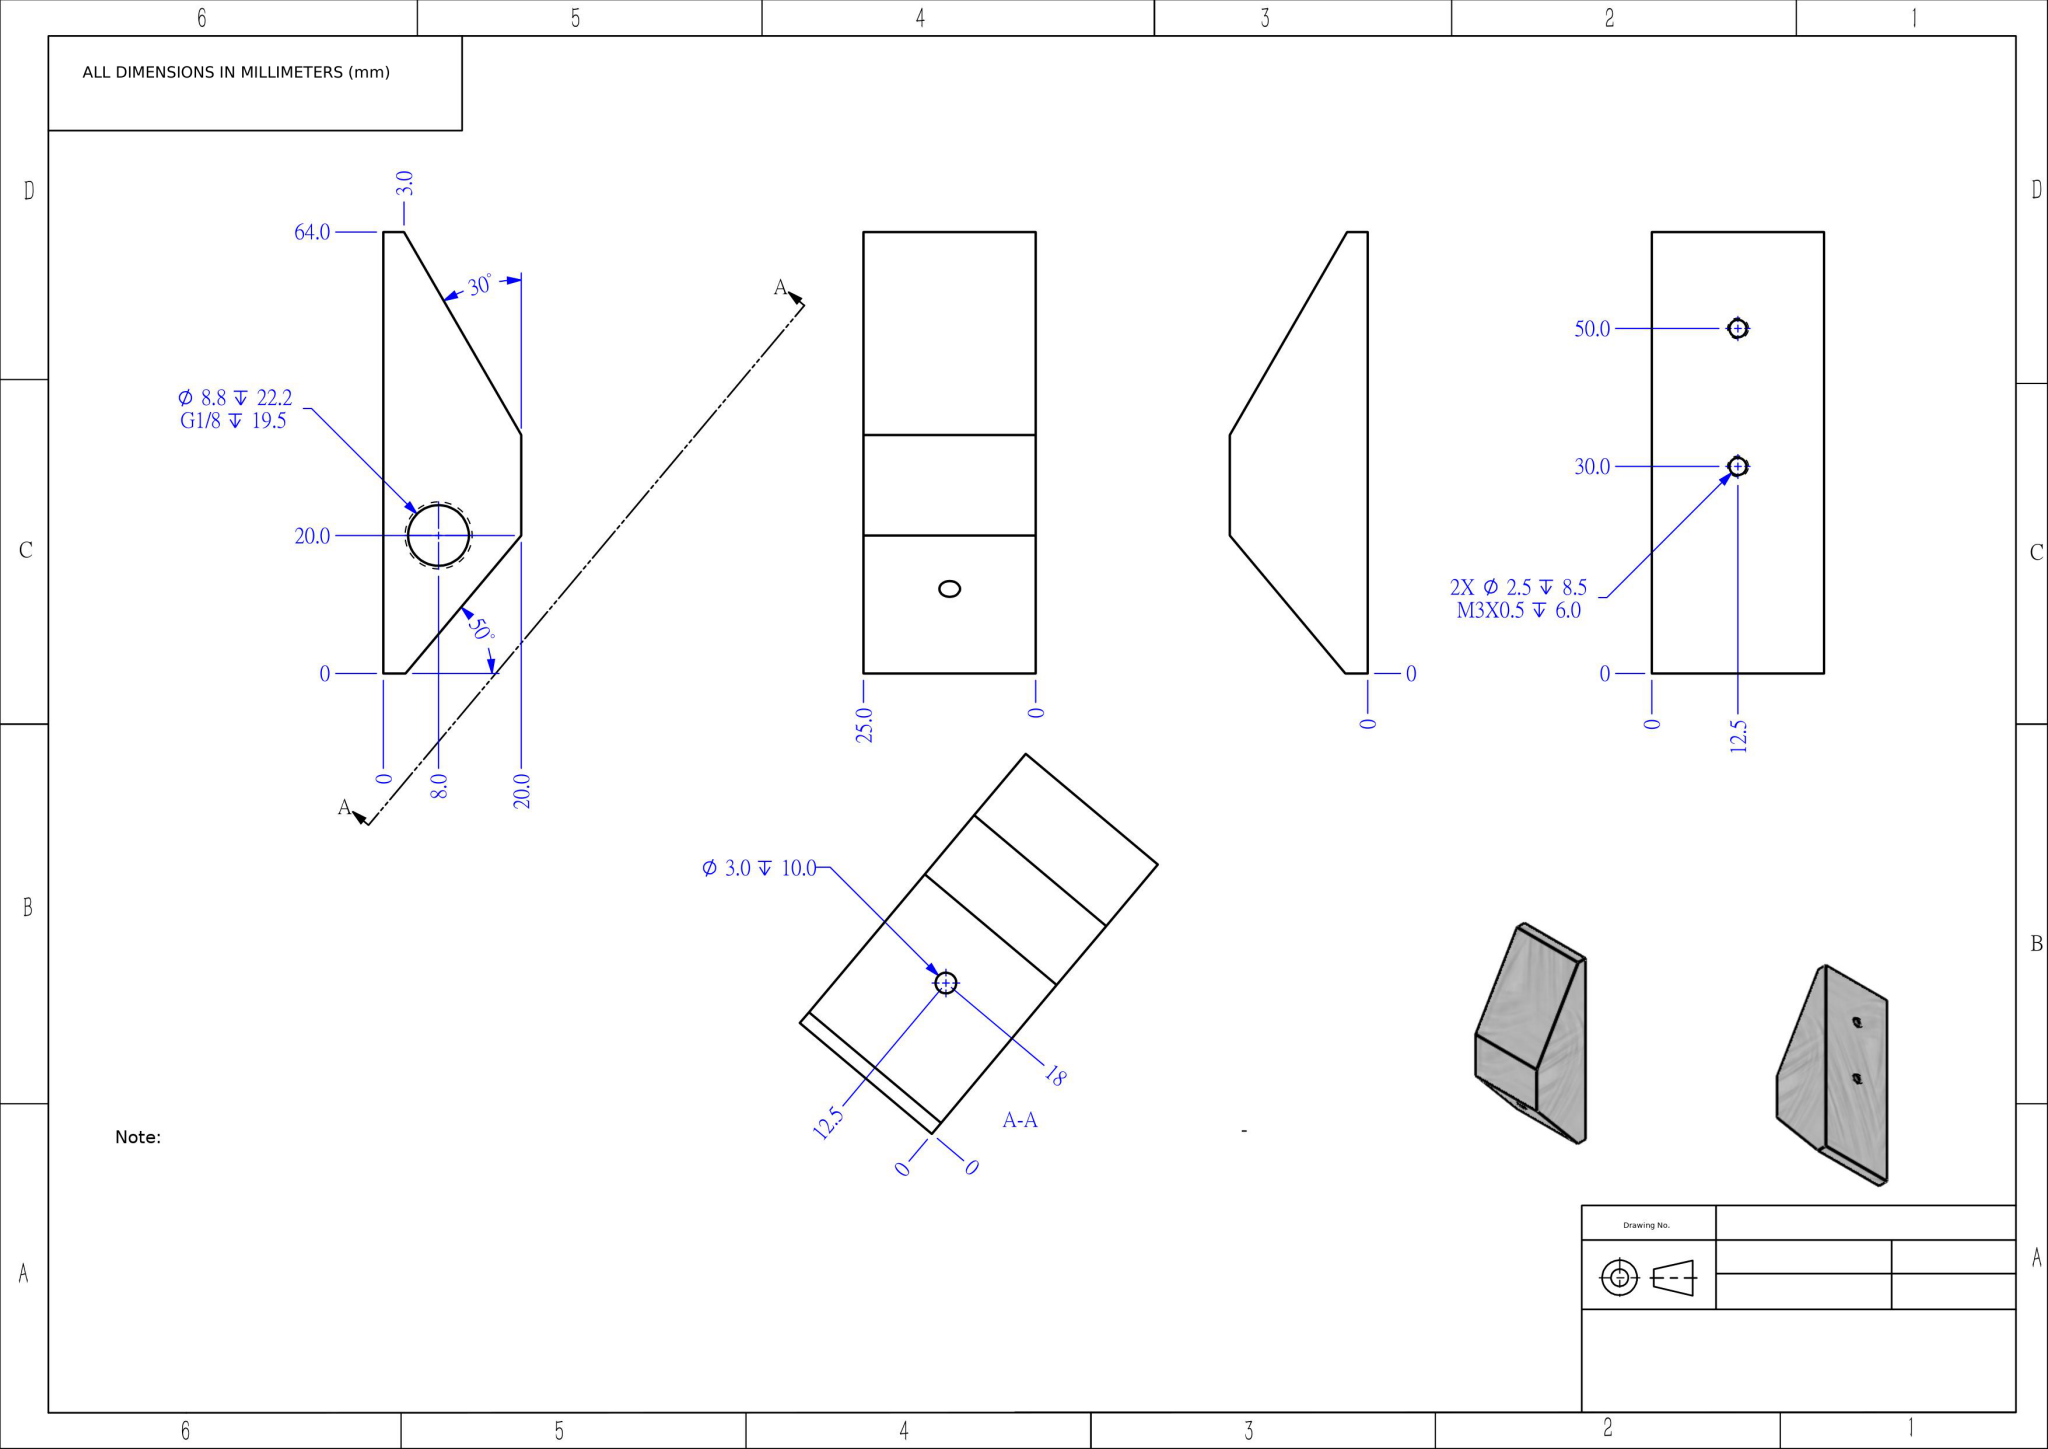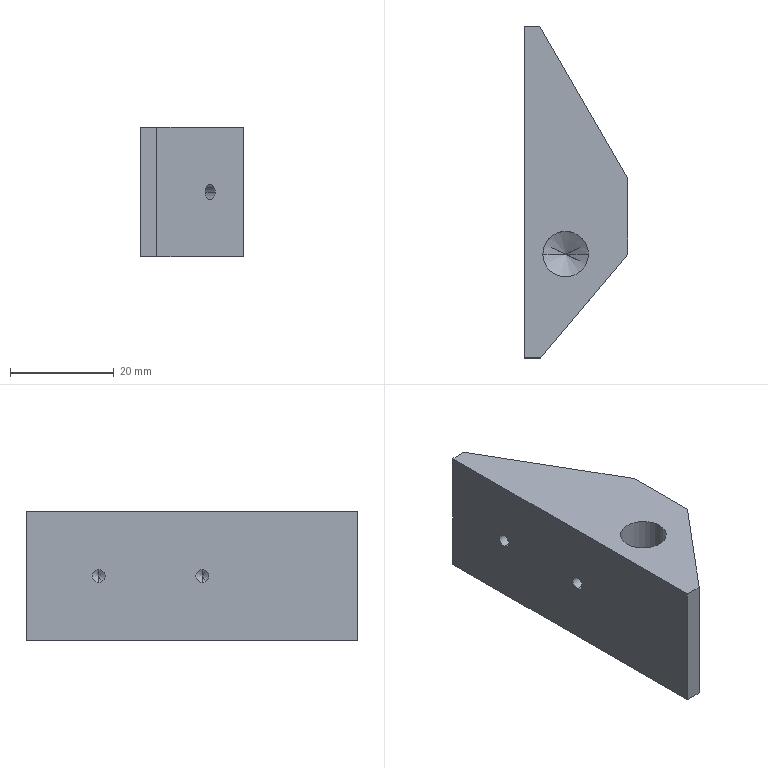Part | NX | mm | 1 solid | 22 faces | box 20 x 64 x 25 mm | volume 20019 mm3 | cylinder 8 | plane 8 | cone 6 | commonest cylinder face diameters 2.5 x4 8.8 x2 3 x2
STEP:
#1=COLOUR_RGB('',1.,1.,1.);
#2=FILL_AREA_STYLE_COLOUR('',#1);
#3=FILL_AREA_STYLE('',(#2));
#4=SURFACE_STYLE_FILL_AREA(#3);
#5=SURFACE_SIDE_STYLE('',(#4));
#6=SURFACE_STYLE_USAGE(.BOTH.,#5);
#7=PRESENTATION_STYLE_ASSIGNMENT((#6));
#8=CARTESIAN_POINT('',(-1.5,18.,11.25));
#9=VERTEX_POINT('',#8);
#10=CARTESIAN_POINT('',(-1.5,18.,13.75));
#11=VERTEX_POINT('',#10);
#12=CARTESIAN_POINT('',(-1.5,18.,12.5));
#13=DIRECTION('',(-1.,0.,0.));
#14=DIRECTION('',(0.,0.,1.));
#15=AXIS2_PLACEMENT_3D('',#12,#13,#14);
#16=CIRCLE('',#15,1.25);
#17=EDGE_CURVE('',#9,#11,#16,.T.);
#18=ORIENTED_EDGE('',*,*,#17,.F.);
#19=CARTESIAN_POINT('',(-10.,18.,11.25));
#20=VERTEX_POINT('',#19);
#21=CARTESIAN_POINT('',(-10.,18.,11.25));
#22=DIRECTION('',(-1.,0.,0.));
#23=VECTOR('',#22,1000.);
#24=LINE('',#21,#23);
#25=EDGE_CURVE('',#9,#20,#24,.T.);
#26=ORIENTED_EDGE('',*,*,#25,.T.);
#27=CARTESIAN_POINT('',(-10.,18.,13.75));
#28=VERTEX_POINT('',#27);
#29=CARTESIAN_POINT('',(-10.,18.,12.5));
#30=DIRECTION('',(-1.,0.,0.));
#31=DIRECTION('',(0.,0.,1.));
#32=AXIS2_PLACEMENT_3D('',#29,#30,#31);
#33=CIRCLE('',#32,1.25);
#34=EDGE_CURVE('',#20,#28,#33,.T.);
#35=ORIENTED_EDGE('',*,*,#34,.T.);
#36=CARTESIAN_POINT('',(-10.,18.,13.75));
#37=DIRECTION('',(-1.,0.,0.));
#38=VECTOR('',#37,1000.);
#39=LINE('',#36,#38);
#40=EDGE_CURVE('',#11,#28,#39,.T.);
#41=ORIENTED_EDGE('',*,*,#40,.F.);
#42=EDGE_LOOP('',(#18,#26,#35,#41));
#43=FACE_OUTER_BOUND('',#42,.T.);
#44=CARTESIAN_POINT('',(-10.,18.,12.5));
#45=DIRECTION('',(-1.,0.,0.));
#46=DIRECTION('',(0.,0.,1.));
#47=AXIS2_PLACEMENT_3D('',#44,#45,#46);
#48=CYLINDRICAL_SURFACE('',#47,1.25);
#49=ADVANCED_FACE('',(#43),#48,.F.);
#50=CARTESIAN_POINT('',(-0.7489,18.,12.5));
#51=VERTEX_POINT('',#50);
#52=CARTESIAN_POINT('',(-1.5,18.,13.75));
#53=DIRECTION('',(-0.515,0.,0.8572));
#54=VECTOR('',#53,1000.);
#55=LINE('',#52,#54);
#56=EDGE_CURVE('',#51,#11,#55,.T.);
#57=ORIENTED_EDGE('',*,*,#56,.F.);
#58=CARTESIAN_POINT('',(-1.5,18.,11.25));
#59=DIRECTION('',(-0.515,0.,-0.8572));
#60=VECTOR('',#59,1000.);
#61=LINE('',#58,#60);
#62=EDGE_CURVE('',#51,#9,#61,.T.);
#63=ORIENTED_EDGE('',*,*,#62,.T.);
#64=ORIENTED_EDGE('',*,*,#17,.T.);
#65=EDGE_LOOP('',(#57,#63,#64));
#66=FACE_OUTER_BOUND('',#65,.T.);
#67=CARTESIAN_POINT('',(-1.5,18.,12.5));
#68=DIRECTION('',(-1.,0.,0.));
#69=DIRECTION('',(0.,0.,1.));
#70=AXIS2_PLACEMENT_3D('',#67,#68,#69);
#71=CONICAL_SURFACE('',#70,1.25,1.03);
#72=ADVANCED_FACE('',(#66),#71,.F.);
#73=CARTESIAN_POINT('',(-1.5,-2.,11.25));
#74=VERTEX_POINT('',#73);
#75=CARTESIAN_POINT('',(-1.5,-2.,13.75));
#76=VERTEX_POINT('',#75);
#77=CARTESIAN_POINT('',(-1.5,-2.,12.5));
#78=DIRECTION('',(-1.,0.,0.));
#79=DIRECTION('',(0.,0.,1.));
#80=AXIS2_PLACEMENT_3D('',#77,#78,#79);
#81=CIRCLE('',#80,1.25);
#82=EDGE_CURVE('',#74,#76,#81,.T.);
#83=ORIENTED_EDGE('',*,*,#82,.F.);
#84=CARTESIAN_POINT('',(-10.,-2.,11.25));
#85=VERTEX_POINT('',#84);
#86=CARTESIAN_POINT('',(-10.,-2.,11.25));
#87=DIRECTION('',(-1.,0.,0.));
#88=VECTOR('',#87,1000.);
#89=LINE('',#86,#88);
#90=EDGE_CURVE('',#74,#85,#89,.T.);
#91=ORIENTED_EDGE('',*,*,#90,.T.);
#92=CARTESIAN_POINT('',(-10.,-2.,13.75));
#93=VERTEX_POINT('',#92);
#94=CARTESIAN_POINT('',(-10.,-2.,12.5));
#95=DIRECTION('',(-1.,0.,0.));
#96=DIRECTION('',(0.,0.,1.));
#97=AXIS2_PLACEMENT_3D('',#94,#95,#96);
#98=CIRCLE('',#97,1.25);
#99=EDGE_CURVE('',#85,#93,#98,.T.);
#100=ORIENTED_EDGE('',*,*,#99,.T.);
#101=CARTESIAN_POINT('',(-10.,-2.,13.75));
#102=DIRECTION('',(-1.,0.,0.));
#103=VECTOR('',#102,1000.);
#104=LINE('',#101,#103);
#105=EDGE_CURVE('',#76,#93,#104,.T.);
#106=ORIENTED_EDGE('',*,*,#105,.F.);
#107=EDGE_LOOP('',(#83,#91,#100,#106));
#108=FACE_OUTER_BOUND('',#107,.T.);
#109=CARTESIAN_POINT('',(-10.,-2.,12.5));
#110=DIRECTION('',(-1.,0.,0.));
#111=DIRECTION('',(0.,0.,1.));
#112=AXIS2_PLACEMENT_3D('',#109,#110,#111);
#113=CYLINDRICAL_SURFACE('',#112,1.25);
#114=ADVANCED_FACE('',(#108),#113,.F.);
#115=CARTESIAN_POINT('',(-0.7489,-2.,12.5));
#116=VERTEX_POINT('',#115);
#117=CARTESIAN_POINT('',(-1.5,-2.,13.75));
#118=DIRECTION('',(-0.515,0.,0.8572));
#119=VECTOR('',#118,1000.);
#120=LINE('',#117,#119);
#121=EDGE_CURVE('',#116,#76,#120,.T.);
#122=ORIENTED_EDGE('',*,*,#121,.F.);
#123=CARTESIAN_POINT('',(-1.5,-2.,11.25));
#124=DIRECTION('',(-0.515,0.,-0.8572));
#125=VECTOR('',#124,1000.);
#126=LINE('',#123,#125);
#127=EDGE_CURVE('',#116,#74,#126,.T.);
#128=ORIENTED_EDGE('',*,*,#127,.T.);
#129=ORIENTED_EDGE('',*,*,#82,.T.);
#130=EDGE_LOOP('',(#122,#128,#129));
#131=FACE_OUTER_BOUND('',#130,.T.);
#132=CARTESIAN_POINT('',(-1.5,-2.,12.5));
#133=DIRECTION('',(-1.,0.,0.));
#134=DIRECTION('',(0.,0.,1.));
#135=AXIS2_PLACEMENT_3D('',#132,#133,#134);
#136=CONICAL_SURFACE('',#135,1.25,1.03);
#137=ADVANCED_FACE('',(#131),#136,.F.);
#138=CARTESIAN_POINT('',(-2.,-12.,0.1792));
#139=VERTEX_POINT('',#138);
#140=CARTESIAN_POINT('',(2.4,-12.,2.823));
#141=VERTEX_POINT('',#140);
#142=CARTESIAN_POINT('',(2.4,-12.,2.823));
#143=DIRECTION('',(0.8572,0.,0.515));
#144=VECTOR('',#143,1000.);
#145=LINE('',#142,#144);
#146=EDGE_CURVE('',#139,#141,#145,.T.);
#147=ORIENTED_EDGE('',*,*,#146,.F.);
#148=CARTESIAN_POINT('',(-6.4,-12.,2.823));
#149=VERTEX_POINT('',#148);
#150=CARTESIAN_POINT('',(-6.4,-12.,2.823));
#151=DIRECTION('',(-0.8572,0.,0.515));
#152=VECTOR('',#151,1000.);
#153=LINE('',#150,#152);
#154=EDGE_CURVE('',#139,#149,#153,.T.);
#155=ORIENTED_EDGE('',*,*,#154,.T.);
#156=CARTESIAN_POINT('',(-2.,-12.,2.823));
#157=DIRECTION('',(0.,0.,1.));
#158=DIRECTION('',(1.,0.,0.));
#159=AXIS2_PLACEMENT_3D('',#156,#157,#158);
#160=CIRCLE('',#159,4.4);
#161=EDGE_CURVE('',#149,#141,#160,.T.);
#162=ORIENTED_EDGE('',*,*,#161,.T.);
#163=EDGE_LOOP('',(#147,#155,#162));
#164=FACE_OUTER_BOUND('',#163,.T.);
#165=CARTESIAN_POINT('',(-2.,-12.,2.823));
#166=DIRECTION('',(0.,0.,1.));
#167=DIRECTION('',(1.,0.,0.));
#168=AXIS2_PLACEMENT_3D('',#165,#166,#167);
#169=CONICAL_SURFACE('',#168,4.4,1.03);
#170=ADVANCED_FACE('',(#164),#169,.F.);
#171=CARTESIAN_POINT('',(0.7251,-15.455,12.5));
#172=VERTEX_POINT('',#171);
#173=CARTESIAN_POINT('',(-2.935,-16.299,12.5));
#174=VERTEX_POINT('',#173);
#175=CARTESIAN_POINT('',(0.7251,-15.455,12.5));
#176=CARTESIAN_POINT('',(0.7251,-15.455,12.387));
#177=CARTESIAN_POINT('',(0.715,-15.463,12.276));
#178=CARTESIAN_POINT('',(0.6748,-15.494,12.058));
#179=CARTESIAN_POINT('',(0.6441,-15.517,11.95));
#180=CARTESIAN_POINT('',(0.5241,-15.605,11.649));
#181=CARTESIAN_POINT('',(0.4035,-15.69,11.471));
#182=CARTESIAN_POINT('',(0.1742,-15.826,11.267));
#183=CARTESIAN_POINT('',(0.08867,-15.874,11.208));
#184=CARTESIAN_POINT('',(-0.09207,-15.966,11.114));
#185=CARTESIAN_POINT('',(-0.1889,-16.011,11.077));
#186=CARTESIAN_POINT('',(-0.492,-16.139,10.999));
#187=CARTESIAN_POINT('',(-0.708,-16.212,10.989));
#188=CARTESIAN_POINT('',(-1.14,-16.321,11.033));
#189=CARTESIAN_POINT('',(-1.359,-16.358,11.087));
#190=CARTESIAN_POINT('',(-1.777,-16.399,11.241));
#191=CARTESIAN_POINT('',(-1.981,-16.404,11.341));
#192=CARTESIAN_POINT('',(-2.357,-16.39,11.581));
#193=CARTESIAN_POINT('',(-2.531,-16.37,11.72));
#194=CARTESIAN_POINT('',(-2.75,-16.336,11.977));
#195=CARTESIAN_POINT('',(-2.814,-16.324,12.071));
#196=CARTESIAN_POINT('',(-2.884,-16.31,12.225));
#197=CARTESIAN_POINT('',(-2.903,-16.306,12.277));
#198=CARTESIAN_POINT('',(-2.928,-16.301,12.386));
#199=CARTESIAN_POINT('',(-2.935,-16.299,12.444));
#200=CARTESIAN_POINT('',(-2.935,-16.299,12.5));
#201=B_SPLINE_CURVE_WITH_KNOTS('',3,(#175,#176,#177,#178,#179,#180,#181,#182,#183,#184,#185,#186,#187,#188,#189,#190,#191,#192,#193,#194,#195,#196,#197,#198,#199,#200),.UNSPECIFIED.,.F.,.F.,(4,2,2,2,2,2,2,2,2,2,2,2,4),(0.,0.0003351,0.0006703,0.001341,0.001676,0.002011,0.002681,0.003351,0.004022,0.004692,0.005027,0.005194,0.005362),.UNSPECIFIED.);
#202=EDGE_CURVE('',#172,#174,#201,.T.);
#203=ORIENTED_EDGE('',*,*,#202,.F.);
#204=CARTESIAN_POINT('',(-2.935,-16.299,12.5));
#205=CARTESIAN_POINT('',(-2.935,-16.299,12.612));
#206=CARTESIAN_POINT('',(-2.907,-16.306,12.725));
#207=CARTESIAN_POINT('',(-2.814,-16.324,12.928));
#208=CARTESIAN_POINT('',(-2.75,-16.336,13.022));
#209=CARTESIAN_POINT('',(-2.534,-16.37,13.278));
#210=CARTESIAN_POINT('',(-2.356,-16.39,13.42));
#211=CARTESIAN_POINT('',(-1.98,-16.404,13.66));
#212=CARTESIAN_POINT('',(-1.778,-16.399,13.759));
#213=CARTESIAN_POINT('',(-1.358,-16.358,13.913));
#214=CARTESIAN_POINT('',(-1.145,-16.322,13.966));
#215=CARTESIAN_POINT('',(-0.8213,-16.241,14.));
#216=CARTESIAN_POINT('',(-0.7117,-16.209,14.003));
#217=CARTESIAN_POINT('',(-0.4994,-16.138,13.991));
#218=CARTESIAN_POINT('',(-0.3956,-16.099,13.976));
#219=CARTESIAN_POINT('',(-0.09186,-15.971,13.898));
#220=CARTESIAN_POINT('',(0.09184,-15.875,13.805));
#221=CARTESIAN_POINT('',(0.3245,-15.737,13.599));
#222=CARTESIAN_POINT('',(0.3927,-15.693,13.522));
#223=CARTESIAN_POINT('',(0.5117,-15.613,13.35));
#224=CARTESIAN_POINT('',(0.5627,-15.577,13.253));
#225=CARTESIAN_POINT('',(0.6836,-15.488,12.952));
#226=CARTESIAN_POINT('',(0.7251,-15.455,12.726));
#227=CARTESIAN_POINT('',(0.7251,-15.455,12.5));
#228=B_SPLINE_CURVE_WITH_KNOTS('',3,(#204,#205,#206,#207,#208,#209,#210,#211,#212,#213,#214,#215,#216,#217,#218,#219,#220,#221,#222,#223,#224,#225,#226,#227),.UNSPECIFIED.,.F.,.F.,(4,2,2,2,2,2,2,2,2,2,2,4),(0.005362,0.005697,0.006032,0.006701,0.007371,0.00804,0.008375,0.00871,0.00938,0.009714,0.01005,0.01072),.UNSPECIFIED.);
#229=EDGE_CURVE('',#174,#172,#228,.T.);
#230=ORIENTED_EDGE('',*,*,#229,.F.);
#231=EDGE_LOOP('',(#203,#230));
#232=FACE_BOUND('',#231,.T.);
#233=ORIENTED_EDGE('',*,*,#161,.F.);
#234=CARTESIAN_POINT('',(-6.4,-12.,25.));
#235=VERTEX_POINT('',#234);
#236=CARTESIAN_POINT('',(-6.4,-12.,25.));
#237=DIRECTION('',(0.,0.,1.));
#238=VECTOR('',#237,1000.);
#239=LINE('',#236,#238);
#240=EDGE_CURVE('',#149,#235,#239,.T.);
#241=ORIENTED_EDGE('',*,*,#240,.T.);
#242=CARTESIAN_POINT('',(2.4,-12.,25.));
#243=VERTEX_POINT('',#242);
#244=CARTESIAN_POINT('',(-2.,-12.,25.));
#245=DIRECTION('',(0.,0.,1.));
#246=DIRECTION('',(1.,0.,0.));
#247=AXIS2_PLACEMENT_3D('',#244,#245,#246);
#248=CIRCLE('',#247,4.4);
#249=EDGE_CURVE('',#235,#243,#248,.T.);
#250=ORIENTED_EDGE('',*,*,#249,.T.);
#251=CARTESIAN_POINT('',(2.4,-12.,25.));
#252=DIRECTION('',(0.,0.,1.));
#253=VECTOR('',#252,1000.);
#254=LINE('',#251,#253);
#255=EDGE_CURVE('',#141,#243,#254,.T.);
#256=ORIENTED_EDGE('',*,*,#255,.F.);
#257=EDGE_LOOP('',(#233,#241,#250,#256));
#258=FACE_OUTER_BOUND('',#257,.T.);
#259=CARTESIAN_POINT('',(-2.,-12.,25.));
#260=DIRECTION('',(0.,0.,1.));
#261=DIRECTION('',(1.,0.,0.));
#262=AXIS2_PLACEMENT_3D('',#259,#260,#261);
#263=CYLINDRICAL_SURFACE('',#262,4.4);
#264=ADVANCED_FACE('',(#232,#258),#263,.F.);
#265=ORIENTED_EDGE('',*,*,#202,.T.);
#266=CARTESIAN_POINT('',(2.538,-20.892,12.5));
#267=VERTEX_POINT('',#266);
#268=CARTESIAN_POINT('',(2.538,-20.892,12.5));
#269=DIRECTION('',(0.766,-0.6428,0.));
#270=VECTOR('',#269,1000.);
#271=LINE('',#268,#270);
#272=EDGE_CURVE('',#174,#267,#271,.T.);
#273=ORIENTED_EDGE('',*,*,#272,.T.);
#274=CARTESIAN_POINT('',(4.467,-18.594,12.5));
#275=VERTEX_POINT('',#274);
#276=CARTESIAN_POINT('',(3.503,-19.743,12.5));
#277=DIRECTION('',(0.766,-0.6428,0.));
#278=DIRECTION('',(0.6428,0.766,0.));
#279=AXIS2_PLACEMENT_3D('',#276,#277,#278);
#280=CIRCLE('',#279,1.5);
#281=EDGE_CURVE('',#267,#275,#280,.T.);
#282=ORIENTED_EDGE('',*,*,#281,.T.);
#283=CARTESIAN_POINT('',(4.467,-18.594,12.5));
#284=DIRECTION('',(0.766,-0.6428,0.));
#285=VECTOR('',#284,1000.);
#286=LINE('',#283,#285);
#287=EDGE_CURVE('',#172,#275,#286,.T.);
#288=ORIENTED_EDGE('',*,*,#287,.F.);
#289=EDGE_LOOP('',(#265,#273,#282,#288));
#290=FACE_OUTER_BOUND('',#289,.T.);
#291=CARTESIAN_POINT('',(3.503,-19.743,12.5));
#292=DIRECTION('',(0.766,-0.6428,0.));
#293=DIRECTION('',(0.6428,0.766,0.));
#294=AXIS2_PLACEMENT_3D('',#291,#292,#293);
#295=CYLINDRICAL_SURFACE('',#294,1.5);
#296=ADVANCED_FACE('',(#290),#295,.F.);
#297=CARTESIAN_POINT('',(10.,-12.,0.));
#298=VERTEX_POINT('',#297);
#299=CARTESIAN_POINT('',(10.,2.555,0.));
#300=VERTEX_POINT('',#299);
#301=CARTESIAN_POINT('',(10.,-32.,0.));
#302=DIRECTION('',(0.,1.,0.));
#303=VECTOR('',#302,1000.);
#304=LINE('',#301,#303);
#305=EDGE_CURVE('',#298,#300,#304,.T.);
#306=ORIENTED_EDGE('',*,*,#305,.T.);
#307=CARTESIAN_POINT('',(10.,2.555,25.));
#308=VERTEX_POINT('',#307);
#309=CARTESIAN_POINT('',(10.,2.555,0.));
#310=DIRECTION('',(0.,0.,1.));
#311=VECTOR('',#310,1000.);
#312=LINE('',#309,#311);
#313=EDGE_CURVE('',#300,#308,#312,.T.);
#314=ORIENTED_EDGE('',*,*,#313,.T.);
#315=CARTESIAN_POINT('',(10.,-12.,25.));
#316=VERTEX_POINT('',#315);
#317=CARTESIAN_POINT('',(10.,-32.,25.));
#318=DIRECTION('',(0.,1.,0.));
#319=VECTOR('',#318,1000.);
#320=LINE('',#317,#319);
#321=EDGE_CURVE('',#316,#308,#320,.T.);
#322=ORIENTED_EDGE('',*,*,#321,.F.);
#323=CARTESIAN_POINT('',(10.,-12.,0.));
#324=DIRECTION('',(0.,0.,1.));
#325=VECTOR('',#324,1000.);
#326=LINE('',#323,#325);
#327=EDGE_CURVE('',#298,#316,#326,.T.);
#328=ORIENTED_EDGE('',*,*,#327,.F.);
#329=EDGE_LOOP('',(#306,#314,#322,#328));
#330=FACE_OUTER_BOUND('',#329,.T.);
#331=CARTESIAN_POINT('',(10.,-32.,25.));
#332=DIRECTION('',(-1.,0.,0.));
#333=DIRECTION('',(0.,0.,1.));
#334=AXIS2_PLACEMENT_3D('',#331,#332,#333);
#335=PLANE('',#334);
#336=ADVANCED_FACE('',(#330),#335,.F.);
#337=CARTESIAN_POINT('',(-7.,32.,25.));
#338=VERTEX_POINT('',#337);
#339=CARTESIAN_POINT('',(-10.,32.,25.));
#340=VERTEX_POINT('',#339);
#341=CARTESIAN_POINT('',(-10.,32.,25.));
#342=DIRECTION('',(-1.,0.,0.));
#343=VECTOR('',#342,1000.);
#344=LINE('',#341,#343);
#345=EDGE_CURVE('',#338,#340,#344,.T.);
#346=ORIENTED_EDGE('',*,*,#345,.F.);
#347=CARTESIAN_POINT('',(-7.,32.,0.));
#348=VERTEX_POINT('',#347);
#349=CARTESIAN_POINT('',(-7.,32.,0.));
#350=DIRECTION('',(0.,0.,1.));
#351=VECTOR('',#350,1000.);
#352=LINE('',#349,#351);
#353=EDGE_CURVE('',#348,#338,#352,.T.);
#354=ORIENTED_EDGE('',*,*,#353,.F.);
#355=CARTESIAN_POINT('',(-10.,32.,0.));
#356=VERTEX_POINT('',#355);
#357=CARTESIAN_POINT('',(-10.,32.,0.));
#358=DIRECTION('',(-1.,0.,0.));
#359=VECTOR('',#358,1000.);
#360=LINE('',#357,#359);
#361=EDGE_CURVE('',#348,#356,#360,.T.);
#362=ORIENTED_EDGE('',*,*,#361,.T.);
#363=CARTESIAN_POINT('',(-10.,32.,25.));
#364=DIRECTION('',(0.,0.,-1.));
#365=VECTOR('',#364,1000.);
#366=LINE('',#363,#365);
#367=EDGE_CURVE('',#340,#356,#366,.T.);
#368=ORIENTED_EDGE('',*,*,#367,.F.);
#369=EDGE_LOOP('',(#346,#354,#362,#368));
#370=FACE_OUTER_BOUND('',#369,.T.);
#371=CARTESIAN_POINT('',(-10.,32.,25.));
#372=DIRECTION('',(0.,-1.,0.));
#373=DIRECTION('',(0.,0.,-1.));
#374=AXIS2_PLACEMENT_3D('',#371,#372,#373);
#375=PLANE('',#374);
#376=ADVANCED_FACE('',(#370),#375,.F.);
#377=CARTESIAN_POINT('',(-10.,18.,12.5));
#378=DIRECTION('',(-1.,0.,0.));
#379=DIRECTION('',(0.,0.,1.));
#380=AXIS2_PLACEMENT_3D('',#377,#378,#379);
#381=CIRCLE('',#380,1.25);
#382=EDGE_CURVE('',#28,#20,#381,.T.);
#383=ORIENTED_EDGE('',*,*,#382,.F.);
#384=ORIENTED_EDGE('',*,*,#34,.F.);
#385=EDGE_LOOP('',(#383,#384));
#386=FACE_BOUND('',#385,.T.);
#387=CARTESIAN_POINT('',(-10.,-2.,12.5));
#388=DIRECTION('',(-1.,0.,0.));
#389=DIRECTION('',(0.,0.,1.));
#390=AXIS2_PLACEMENT_3D('',#387,#388,#389);
#391=CIRCLE('',#390,1.25);
#392=EDGE_CURVE('',#93,#85,#391,.T.);
#393=ORIENTED_EDGE('',*,*,#392,.F.);
#394=ORIENTED_EDGE('',*,*,#99,.F.);
#395=EDGE_LOOP('',(#393,#394));
#396=FACE_BOUND('',#395,.T.);
#397=CARTESIAN_POINT('',(-10.,-32.,0.));
#398=VERTEX_POINT('',#397);
#399=CARTESIAN_POINT('',(-10.,-32.,0.));
#400=DIRECTION('',(0.,-1.,0.));
#401=VECTOR('',#400,1000.);
#402=LINE('',#399,#401);
#403=EDGE_CURVE('',#356,#398,#402,.T.);
#404=ORIENTED_EDGE('',*,*,#403,.T.);
#405=CARTESIAN_POINT('',(-10.,-32.,25.));
#406=VERTEX_POINT('',#405);
#407=CARTESIAN_POINT('',(-10.,-32.,25.));
#408=DIRECTION('',(0.,0.,-1.));
#409=VECTOR('',#408,1000.);
#410=LINE('',#407,#409);
#411=EDGE_CURVE('',#406,#398,#410,.T.);
#412=ORIENTED_EDGE('',*,*,#411,.F.);
#413=CARTESIAN_POINT('',(-10.,-32.,25.));
#414=DIRECTION('',(0.,-1.,0.));
#415=VECTOR('',#414,1000.);
#416=LINE('',#413,#415);
#417=EDGE_CURVE('',#340,#406,#416,.T.);
#418=ORIENTED_EDGE('',*,*,#417,.F.);
#419=ORIENTED_EDGE('',*,*,#367,.T.);
#420=EDGE_LOOP('',(#404,#412,#418,#419));
#421=FACE_OUTER_BOUND('',#420,.T.);
#422=CARTESIAN_POINT('',(-10.,-32.,25.));
#423=DIRECTION('',(1.,0.,0.));
#424=DIRECTION('',(0.,0.,-1.));
#425=AXIS2_PLACEMENT_3D('',#422,#423,#424);
#426=PLANE('',#425);
#427=ADVANCED_FACE('',(#386,#396,#421),#426,.F.);
#428=CARTESIAN_POINT('',(-6.782,-32.,0.));
#429=VERTEX_POINT('',#428);
#430=CARTESIAN_POINT('',(-10.,-32.,0.));
#431=DIRECTION('',(1.,0.,0.));
#432=VECTOR('',#431,1000.);
#433=LINE('',#430,#432);
#434=EDGE_CURVE('',#398,#429,#433,.T.);
#435=ORIENTED_EDGE('',*,*,#434,.T.);
#436=CARTESIAN_POINT('',(-6.782,-32.,25.));
#437=VERTEX_POINT('',#436);
#438=CARTESIAN_POINT('',(-6.782,-32.,0.));
#439=DIRECTION('',(0.,0.,1.));
#440=VECTOR('',#439,1000.);
#441=LINE('',#438,#440);
#442=EDGE_CURVE('',#429,#437,#441,.T.);
#443=ORIENTED_EDGE('',*,*,#442,.T.);
#444=CARTESIAN_POINT('',(-10.,-32.,25.));
#445=DIRECTION('',(1.,0.,0.));
#446=VECTOR('',#445,1000.);
#447=LINE('',#444,#446);
#448=EDGE_CURVE('',#406,#437,#447,.T.);
#449=ORIENTED_EDGE('',*,*,#448,.F.);
#450=ORIENTED_EDGE('',*,*,#411,.T.);
#451=EDGE_LOOP('',(#435,#443,#449,#450));
#452=FACE_OUTER_BOUND('',#451,.T.);
#453=CARTESIAN_POINT('',(-10.,-32.,25.));
#454=DIRECTION('',(0.,1.,0.));
#455=DIRECTION('',(0.,0.,1.));
#456=AXIS2_PLACEMENT_3D('',#453,#454,#455);
#457=PLANE('',#456);
#458=ADVANCED_FACE('',(#452),#457,.F.);
#459=CARTESIAN_POINT('',(-2.,-12.,25.));
#460=DIRECTION('',(0.,0.,1.));
#461=DIRECTION('',(1.,0.,0.));
#462=AXIS2_PLACEMENT_3D('',#459,#460,#461);
#463=CIRCLE('',#462,4.4);
#464=EDGE_CURVE('',#243,#235,#463,.T.);
#465=ORIENTED_EDGE('',*,*,#464,.F.);
#466=ORIENTED_EDGE('',*,*,#249,.F.);
#467=EDGE_LOOP('',(#465,#466));
#468=FACE_BOUND('',#467,.T.);
#469=ORIENTED_EDGE('',*,*,#321,.T.);
#470=CARTESIAN_POINT('',(-7.,32.,25.));
#471=DIRECTION('',(0.5,-0.866,0.));
#472=VECTOR('',#471,1000.);
#473=LINE('',#470,#472);
#474=EDGE_CURVE('',#338,#308,#473,.T.);
#475=ORIENTED_EDGE('',*,*,#474,.F.);
#476=ORIENTED_EDGE('',*,*,#345,.T.);
#477=ORIENTED_EDGE('',*,*,#417,.T.);
#478=ORIENTED_EDGE('',*,*,#448,.T.);
#479=CARTESIAN_POINT('',(10.,-12.,25.));
#480=DIRECTION('',(-0.6428,-0.766,0.));
#481=VECTOR('',#480,1000.);
#482=LINE('',#479,#481);
#483=EDGE_CURVE('',#316,#437,#482,.T.);
#484=ORIENTED_EDGE('',*,*,#483,.F.);
#485=EDGE_LOOP('',(#469,#475,#476,#477,#478,#484));
#486=FACE_OUTER_BOUND('',#485,.T.);
#487=CARTESIAN_POINT('',(0.,0.,25.));
#488=DIRECTION('',(0.,0.,-1.));
#489=DIRECTION('',(-1.,0.,0.));
#490=AXIS2_PLACEMENT_3D('',#487,#488,#489);
#491=PLANE('',#490);
#492=ADVANCED_FACE('',(#468,#486),#491,.F.);
#493=CARTESIAN_POINT('',(-7.,32.,0.));
#494=DIRECTION('',(0.5,-0.866,0.));
#495=VECTOR('',#494,1000.);
#496=LINE('',#493,#495);
#497=EDGE_CURVE('',#348,#300,#496,.T.);
#498=ORIENTED_EDGE('',*,*,#497,.T.);
#499=ORIENTED_EDGE('',*,*,#305,.F.);
#500=CARTESIAN_POINT('',(10.,-12.,0.));
#501=DIRECTION('',(-0.6428,-0.766,0.));
#502=VECTOR('',#501,1000.);
#503=LINE('',#500,#502);
#504=EDGE_CURVE('',#298,#429,#503,.T.);
#505=ORIENTED_EDGE('',*,*,#504,.T.);
#506=ORIENTED_EDGE('',*,*,#434,.F.);
#507=ORIENTED_EDGE('',*,*,#403,.F.);
#508=ORIENTED_EDGE('',*,*,#361,.F.);
#509=EDGE_LOOP('',(#498,#499,#505,#506,#507,#508));
#510=FACE_OUTER_BOUND('',#509,.T.);
#511=CARTESIAN_POINT('',(0.,0.,0.));
#512=DIRECTION('',(0.,0.,-1.));
#513=DIRECTION('',(-1.,0.,0.));
#514=AXIS2_PLACEMENT_3D('',#511,#512,#513);
#515=PLANE('',#514);
#516=ADVANCED_FACE('',(#510),#515,.T.);
#517=CARTESIAN_POINT('',(3.503,-19.743,12.5));
#518=DIRECTION('',(0.766,-0.6428,0.));
#519=DIRECTION('',(0.6428,0.766,0.));
#520=AXIS2_PLACEMENT_3D('',#517,#518,#519);
#521=CIRCLE('',#520,1.5);
#522=EDGE_CURVE('',#275,#267,#521,.T.);
#523=ORIENTED_EDGE('',*,*,#522,.F.);
#524=ORIENTED_EDGE('',*,*,#281,.F.);
#525=EDGE_LOOP('',(#523,#524));
#526=FACE_BOUND('',#525,.T.);
#527=ORIENTED_EDGE('',*,*,#483,.T.);
#528=ORIENTED_EDGE('',*,*,#442,.F.);
#529=ORIENTED_EDGE('',*,*,#504,.F.);
#530=ORIENTED_EDGE('',*,*,#327,.T.);
#531=EDGE_LOOP('',(#527,#528,#529,#530));
#532=FACE_OUTER_BOUND('',#531,.T.);
#533=CARTESIAN_POINT('',(10.,-12.,0.));
#534=DIRECTION('',(-0.766,0.6428,0.));
#535=DIRECTION('',(-0.6428,-0.766,0.));
#536=AXIS2_PLACEMENT_3D('',#533,#534,#535);
#537=PLANE('',#536);
#538=ADVANCED_FACE('',(#526,#532),#537,.F.);
#539=ORIENTED_EDGE('',*,*,#474,.T.);
#540=ORIENTED_EDGE('',*,*,#313,.F.);
#541=ORIENTED_EDGE('',*,*,#497,.F.);
#542=ORIENTED_EDGE('',*,*,#353,.T.);
#543=EDGE_LOOP('',(#539,#540,#541,#542));
#544=FACE_OUTER_BOUND('',#543,.T.);
#545=CARTESIAN_POINT('',(-7.,32.,0.));
#546=DIRECTION('',(-0.866,-0.5,0.));
#547=DIRECTION('',(0.5,-0.866,0.));
#548=AXIS2_PLACEMENT_3D('',#545,#546,#547);
#549=PLANE('',#548);
#550=ADVANCED_FACE('',(#544),#549,.F.);
#551=ORIENTED_EDGE('',*,*,#272,.F.);
#552=ORIENTED_EDGE('',*,*,#229,.T.);
#553=ORIENTED_EDGE('',*,*,#287,.T.);
#554=ORIENTED_EDGE('',*,*,#522,.T.);
#555=EDGE_LOOP('',(#551,#552,#553,#554));
#556=FACE_OUTER_BOUND('',#555,.T.);
#557=CARTESIAN_POINT('',(3.503,-19.743,12.5));
#558=DIRECTION('',(0.766,-0.6428,0.));
#559=DIRECTION('',(0.6428,0.766,0.));
#560=AXIS2_PLACEMENT_3D('',#557,#558,#559);
#561=CYLINDRICAL_SURFACE('',#560,1.5);
#562=ADVANCED_FACE('',(#556),#561,.F.);
#563=ORIENTED_EDGE('',*,*,#240,.F.);
#564=CARTESIAN_POINT('',(-2.,-12.,2.823));
#565=DIRECTION('',(0.,0.,1.));
#566=DIRECTION('',(1.,0.,0.));
#567=AXIS2_PLACEMENT_3D('',#564,#565,#566);
#568=CIRCLE('',#567,4.4);
#569=EDGE_CURVE('',#141,#149,#568,.T.);
#570=ORIENTED_EDGE('',*,*,#569,.F.);
#571=ORIENTED_EDGE('',*,*,#255,.T.);
#572=ORIENTED_EDGE('',*,*,#464,.T.);
#573=EDGE_LOOP('',(#563,#570,#571,#572));
#574=FACE_OUTER_BOUND('',#573,.T.);
#575=CARTESIAN_POINT('',(-2.,-12.,25.));
#576=DIRECTION('',(0.,0.,1.));
#577=DIRECTION('',(1.,0.,0.));
#578=AXIS2_PLACEMENT_3D('',#575,#576,#577);
#579=CYLINDRICAL_SURFACE('',#578,4.4);
#580=ADVANCED_FACE('',(#574),#579,.F.);
#581=ORIENTED_EDGE('',*,*,#154,.F.);
#582=ORIENTED_EDGE('',*,*,#146,.T.);
#583=ORIENTED_EDGE('',*,*,#569,.T.);
#584=EDGE_LOOP('',(#581,#582,#583));
#585=FACE_OUTER_BOUND('',#584,.T.);
#586=CARTESIAN_POINT('',(-2.,-12.,2.823));
#587=DIRECTION('',(0.,0.,1.));
#588=DIRECTION('',(1.,0.,0.));
#589=AXIS2_PLACEMENT_3D('',#586,#587,#588);
#590=CONICAL_SURFACE('',#589,4.4,1.03);
#591=ADVANCED_FACE('',(#585),#590,.F.);
#592=ORIENTED_EDGE('',*,*,#127,.F.);
#593=ORIENTED_EDGE('',*,*,#121,.T.);
#594=CARTESIAN_POINT('',(-1.5,-2.,12.5));
#595=DIRECTION('',(-1.,0.,0.));
#596=DIRECTION('',(0.,0.,1.));
#597=AXIS2_PLACEMENT_3D('',#594,#595,#596);
#598=CIRCLE('',#597,1.25);
#599=EDGE_CURVE('',#76,#74,#598,.T.);
#600=ORIENTED_EDGE('',*,*,#599,.T.);
#601=EDGE_LOOP('',(#592,#593,#600));
#602=FACE_OUTER_BOUND('',#601,.T.);
#603=CARTESIAN_POINT('',(-1.5,-2.,12.5));
#604=DIRECTION('',(-1.,0.,0.));
#605=DIRECTION('',(0.,0.,1.));
#606=AXIS2_PLACEMENT_3D('',#603,#604,#605);
#607=CONICAL_SURFACE('',#606,1.25,1.03);
#608=ADVANCED_FACE('',(#602),#607,.F.);
#609=ORIENTED_EDGE('',*,*,#90,.F.);
#610=ORIENTED_EDGE('',*,*,#599,.F.);
#611=ORIENTED_EDGE('',*,*,#105,.T.);
#612=ORIENTED_EDGE('',*,*,#392,.T.);
#613=EDGE_LOOP('',(#609,#610,#611,#612));
#614=FACE_OUTER_BOUND('',#613,.T.);
#615=CARTESIAN_POINT('',(-10.,-2.,12.5));
#616=DIRECTION('',(-1.,0.,0.));
#617=DIRECTION('',(0.,0.,1.));
#618=AXIS2_PLACEMENT_3D('',#615,#616,#617);
#619=CYLINDRICAL_SURFACE('',#618,1.25);
#620=ADVANCED_FACE('',(#614),#619,.F.);
#621=ORIENTED_EDGE('',*,*,#62,.F.);
#622=ORIENTED_EDGE('',*,*,#56,.T.);
#623=CARTESIAN_POINT('',(-1.5,18.,12.5));
#624=DIRECTION('',(-1.,0.,0.));
#625=DIRECTION('',(0.,0.,1.));
#626=AXIS2_PLACEMENT_3D('',#623,#624,#625);
#627=CIRCLE('',#626,1.25);
#628=EDGE_CURVE('',#11,#9,#627,.T.);
#629=ORIENTED_EDGE('',*,*,#628,.T.);
#630=EDGE_LOOP('',(#621,#622,#629));
#631=FACE_OUTER_BOUND('',#630,.T.);
#632=CARTESIAN_POINT('',(-1.5,18.,12.5));
#633=DIRECTION('',(-1.,0.,0.));
#634=DIRECTION('',(0.,0.,1.));
#635=AXIS2_PLACEMENT_3D('',#632,#633,#634);
#636=CONICAL_SURFACE('',#635,1.25,1.03);
#637=ADVANCED_FACE('',(#631),#636,.F.);
#638=ORIENTED_EDGE('',*,*,#25,.F.);
#639=ORIENTED_EDGE('',*,*,#628,.F.);
#640=ORIENTED_EDGE('',*,*,#40,.T.);
#641=ORIENTED_EDGE('',*,*,#382,.T.);
#642=EDGE_LOOP('',(#638,#639,#640,#641));
#643=FACE_OUTER_BOUND('',#642,.T.);
#644=CARTESIAN_POINT('',(-10.,18.,12.5));
#645=DIRECTION('',(-1.,0.,0.));
#646=DIRECTION('',(0.,0.,1.));
#647=AXIS2_PLACEMENT_3D('',#644,#645,#646);
#648=CYLINDRICAL_SURFACE('',#647,1.25);
#649=ADVANCED_FACE('',(#643),#648,.F.);
#650=CLOSED_SHELL('',(#49,#72,#114,#137,#170,#264,#296,#336,#376,#427,#458,#492,#516,#538,#550,#562,#580,#591,#608,#620,#637,#649));
#651=MANIFOLD_SOLID_BREP('',#650);
#652=STYLED_ITEM('',(#7),#651);
#653=(LENGTH_UNIT()NAMED_UNIT(*)SI_UNIT(.MILLI.,.METRE.));
#654=UNCERTAINTY_MEASURE_WITH_UNIT(LENGTH_MEASURE(0.00001),#653,'','');
#655=(NAMED_UNIT(*)PLANE_ANGLE_UNIT()SI_UNIT($,.RADIAN.));
#656=(NAMED_UNIT(*)SI_UNIT($,.STERADIAN.)SOLID_ANGLE_UNIT());
#657=(GEOMETRIC_REPRESENTATION_CONTEXT(3)GLOBAL_UNCERTAINTY_ASSIGNED_CONTEXT((#654))GLOBAL_UNIT_ASSIGNED_CONTEXT((#653,#655,#656))REPRESENTATION_CONTEXT('',''));
#658=MECHANICAL_DESIGN_GEOMETRIC_PRESENTATION_REPRESENTATION('',(#652),#657);
#659=COLOUR_RGB('',1.,1.,1.);
#660=FILL_AREA_STYLE_COLOUR('',#659);
#661=FILL_AREA_STYLE('',(#660));
#662=SURFACE_STYLE_FILL_AREA(#661);
#663=SURFACE_SIDE_STYLE('',(#662));
#664=SURFACE_STYLE_USAGE(.BOTH.,#663);
#665=PRESENTATION_STYLE_ASSIGNMENT((#664));
#666=STYLED_ITEM('',(#665),#649);
#667=(LENGTH_UNIT()NAMED_UNIT(*)SI_UNIT(.MILLI.,.METRE.));
#668=UNCERTAINTY_MEASURE_WITH_UNIT(LENGTH_MEASURE(0.00001),#667,'','');
#669=(NAMED_UNIT(*)PLANE_ANGLE_UNIT()SI_UNIT($,.RADIAN.));
#670=(NAMED_UNIT(*)SI_UNIT($,.STERADIAN.)SOLID_ANGLE_UNIT());
#671=(GEOMETRIC_REPRESENTATION_CONTEXT(3)GLOBAL_UNCERTAINTY_ASSIGNED_CONTEXT((#668))GLOBAL_UNIT_ASSIGNED_CONTEXT((#667,#669,#670))REPRESENTATION_CONTEXT('',''));
#672=MECHANICAL_DESIGN_GEOMETRIC_PRESENTATION_REPRESENTATION('',(#666),#671);
#673=COLOUR_RGB('',1.,1.,1.);
#674=FILL_AREA_STYLE_COLOUR('',#673);
#675=FILL_AREA_STYLE('',(#674));
#676=SURFACE_STYLE_FILL_AREA(#675);
#677=SURFACE_SIDE_STYLE('',(#676));
#678=SURFACE_STYLE_USAGE(.BOTH.,#677);
#679=PRESENTATION_STYLE_ASSIGNMENT((#678));
#680=STYLED_ITEM('',(#679),#264);
#681=PRESENTATION_LAYER_ASSIGNMENT('','',(#680));
#682=COLOUR_RGB('',1.,1.,1.);
#683=FILL_AREA_STYLE_COLOUR('',#682);
#684=FILL_AREA_STYLE('',(#683));
#685=SURFACE_STYLE_FILL_AREA(#684);
#686=SURFACE_SIDE_STYLE('',(#685));
#687=SURFACE_STYLE_USAGE(.BOTH.,#686);
#688=PRESENTATION_STYLE_ASSIGNMENT((#687));
#689=CARTESIAN_POINT('',(0.,0.,0.));
#690=DIRECTION('',(0.,0.,1.));
#691=DIRECTION('',(1.,0.,0.));
#692=AXIS2_PLACEMENT_3D('',#689,#690,#691);
#693=(LENGTH_UNIT()NAMED_UNIT(*)SI_UNIT(.MILLI.,.METRE.));
#694=UNCERTAINTY_MEASURE_WITH_UNIT(LENGTH_MEASURE(0.00001),#693,'','');
#695=(NAMED_UNIT(*)PLANE_ANGLE_UNIT()SI_UNIT($,.RADIAN.));
#696=(NAMED_UNIT(*)SI_UNIT($,.STERADIAN.)SOLID_ANGLE_UNIT());
#697=(GEOMETRIC_REPRESENTATION_CONTEXT(3)GLOBAL_UNCERTAINTY_ASSIGNED_CONTEXT((#694))GLOBAL_UNIT_ASSIGNED_CONTEXT((#693,#695,#696))REPRESENTATION_CONTEXT('',''));
#698=ADVANCED_BREP_SHAPE_REPRESENTATION('',(#651,#692),#697);
#699=STYLED_ITEM('',(#688),#698);
#700=PRESENTATION_LAYER_ASSIGNMENT('','',(#699));
#701=COLOUR_RGB('',1.,1.,1.);
#702=FILL_AREA_STYLE_COLOUR('',#701);
#703=FILL_AREA_STYLE('',(#702));
#704=SURFACE_STYLE_FILL_AREA(#703);
#705=SURFACE_SIDE_STYLE('',(#704));
#706=SURFACE_STYLE_USAGE(.BOTH.,#705);
#707=PRESENTATION_STYLE_ASSIGNMENT((#706));
#708=STYLED_ITEM('',(#707),#114);
#709=(LENGTH_UNIT()NAMED_UNIT(*)SI_UNIT(.MILLI.,.METRE.));
#710=UNCERTAINTY_MEASURE_WITH_UNIT(LENGTH_MEASURE(0.00001),#709,'','');
#711=(NAMED_UNIT(*)PLANE_ANGLE_UNIT()SI_UNIT($,.RADIAN.));
#712=(NAMED_UNIT(*)SI_UNIT($,.STERADIAN.)SOLID_ANGLE_UNIT());
#713=(GEOMETRIC_REPRESENTATION_CONTEXT(3)GLOBAL_UNCERTAINTY_ASSIGNED_CONTEXT((#710))GLOBAL_UNIT_ASSIGNED_CONTEXT((#709,#711,#712))REPRESENTATION_CONTEXT('',''));
#714=MECHANICAL_DESIGN_GEOMETRIC_PRESENTATION_REPRESENTATION('',(#708),#713);
#715=COLOUR_RGB('',1.,1.,1.);
#716=FILL_AREA_STYLE_COLOUR('',#715);
#717=FILL_AREA_STYLE('',(#716));
#718=SURFACE_STYLE_FILL_AREA(#717);
#719=SURFACE_SIDE_STYLE('',(#718));
#720=SURFACE_STYLE_USAGE(.BOTH.,#719);
#721=PRESENTATION_STYLE_ASSIGNMENT((#720));
#722=STYLED_ITEM('',(#721),#49);
#723=PRESENTATION_LAYER_ASSIGNMENT('','',(#722));
#724=COLOUR_RGB('',1.,1.,1.);
#725=FILL_AREA_STYLE_COLOUR('',#724);
#726=FILL_AREA_STYLE('',(#725));
#727=SURFACE_STYLE_FILL_AREA(#726);
#728=SURFACE_SIDE_STYLE('',(#727));
#729=SURFACE_STYLE_USAGE(.BOTH.,#728);
#730=PRESENTATION_STYLE_ASSIGNMENT((#729));
#731=STYLED_ITEM('',(#730),#620);
#732=(LENGTH_UNIT()NAMED_UNIT(*)SI_UNIT(.MILLI.,.METRE.));
#733=UNCERTAINTY_MEASURE_WITH_UNIT(LENGTH_MEASURE(0.00001),#732,'','');
#734=(NAMED_UNIT(*)PLANE_ANGLE_UNIT()SI_UNIT($,.RADIAN.));
#735=(NAMED_UNIT(*)SI_UNIT($,.STERADIAN.)SOLID_ANGLE_UNIT());
#736=(GEOMETRIC_REPRESENTATION_CONTEXT(3)GLOBAL_UNCERTAINTY_ASSIGNED_CONTEXT((#733))GLOBAL_UNIT_ASSIGNED_CONTEXT((#732,#734,#735))REPRESENTATION_CONTEXT('',''));
#737=MECHANICAL_DESIGN_GEOMETRIC_PRESENTATION_REPRESENTATION('',(#731),#736);
#738=COLOUR_RGB('',1.,1.,1.);
#739=FILL_AREA_STYLE_COLOUR('',#738);
#740=FILL_AREA_STYLE('',(#739));
#741=SURFACE_STYLE_FILL_AREA(#740);
#742=SURFACE_SIDE_STYLE('',(#741));
#743=SURFACE_STYLE_USAGE(.BOTH.,#742);
#744=PRESENTATION_STYLE_ASSIGNMENT((#743));
#745=STYLED_ITEM('',(#744),#580);
#746=PRESENTATION_LAYER_ASSIGNMENT('','',(#745));
#747=PRESENTATION_LAYER_ASSIGNMENT('','',(#652));
#748=PRESENTATION_LAYER_ASSIGNMENT('','',(#666));
#749=PRESENTATION_LAYER_ASSIGNMENT('','',(#708));
#750=PRESENTATION_LAYER_ASSIGNMENT('','',(#731));
#751=(LENGTH_UNIT()NAMED_UNIT(*)SI_UNIT(.MILLI.,.METRE.));
#752=UNCERTAINTY_MEASURE_WITH_UNIT(LENGTH_MEASURE(0.00001),#751,'','');
#753=(NAMED_UNIT(*)PLANE_ANGLE_UNIT()SI_UNIT($,.RADIAN.));
#754=(NAMED_UNIT(*)SI_UNIT($,.STERADIAN.)SOLID_ANGLE_UNIT());
#755=(GEOMETRIC_REPRESENTATION_CONTEXT(3)GLOBAL_UNCERTAINTY_ASSIGNED_CONTEXT((#752))GLOBAL_UNIT_ASSIGNED_CONTEXT((#751,#753,#754))REPRESENTATION_CONTEXT('',''));
#756=MECHANICAL_DESIGN_GEOMETRIC_PRESENTATION_REPRESENTATION('',(#680),#755);
#757=(LENGTH_UNIT()NAMED_UNIT(*)SI_UNIT(.MILLI.,.METRE.));
#758=UNCERTAINTY_MEASURE_WITH_UNIT(LENGTH_MEASURE(0.00001),#757,'','');
#759=(NAMED_UNIT(*)PLANE_ANGLE_UNIT()SI_UNIT($,.RADIAN.));
#760=(NAMED_UNIT(*)SI_UNIT($,.STERADIAN.)SOLID_ANGLE_UNIT());
#761=(GEOMETRIC_REPRESENTATION_CONTEXT(3)GLOBAL_UNCERTAINTY_ASSIGNED_CONTEXT((#758))GLOBAL_UNIT_ASSIGNED_CONTEXT((#757,#759,#760))REPRESENTATION_CONTEXT('',''));
#762=MECHANICAL_DESIGN_GEOMETRIC_PRESENTATION_REPRESENTATION('',(#699),#761);
#763=(LENGTH_UNIT()NAMED_UNIT(*)SI_UNIT(.MILLI.,.METRE.));
#764=UNCERTAINTY_MEASURE_WITH_UNIT(LENGTH_MEASURE(0.00001),#763,'','');
#765=(NAMED_UNIT(*)PLANE_ANGLE_UNIT()SI_UNIT($,.RADIAN.));
#766=(NAMED_UNIT(*)SI_UNIT($,.STERADIAN.)SOLID_ANGLE_UNIT());
#767=(GEOMETRIC_REPRESENTATION_CONTEXT(3)GLOBAL_UNCERTAINTY_ASSIGNED_CONTEXT((#764))GLOBAL_UNIT_ASSIGNED_CONTEXT((#763,#765,#766))REPRESENTATION_CONTEXT('',''));
#768=MECHANICAL_DESIGN_GEOMETRIC_PRESENTATION_REPRESENTATION('',(#722),#767);
#769=(LENGTH_UNIT()NAMED_UNIT(*)SI_UNIT(.MILLI.,.METRE.));
#770=UNCERTAINTY_MEASURE_WITH_UNIT(LENGTH_MEASURE(0.00001),#769,'','');
#771=(NAMED_UNIT(*)PLANE_ANGLE_UNIT()SI_UNIT($,.RADIAN.));
#772=(NAMED_UNIT(*)SI_UNIT($,.STERADIAN.)SOLID_ANGLE_UNIT());
#773=(GEOMETRIC_REPRESENTATION_CONTEXT(3)GLOBAL_UNCERTAINTY_ASSIGNED_CONTEXT((#770))GLOBAL_UNIT_ASSIGNED_CONTEXT((#769,#771,#772))REPRESENTATION_CONTEXT('',''));
#774=MECHANICAL_DESIGN_GEOMETRIC_PRESENTATION_REPRESENTATION('',(#745),#773);